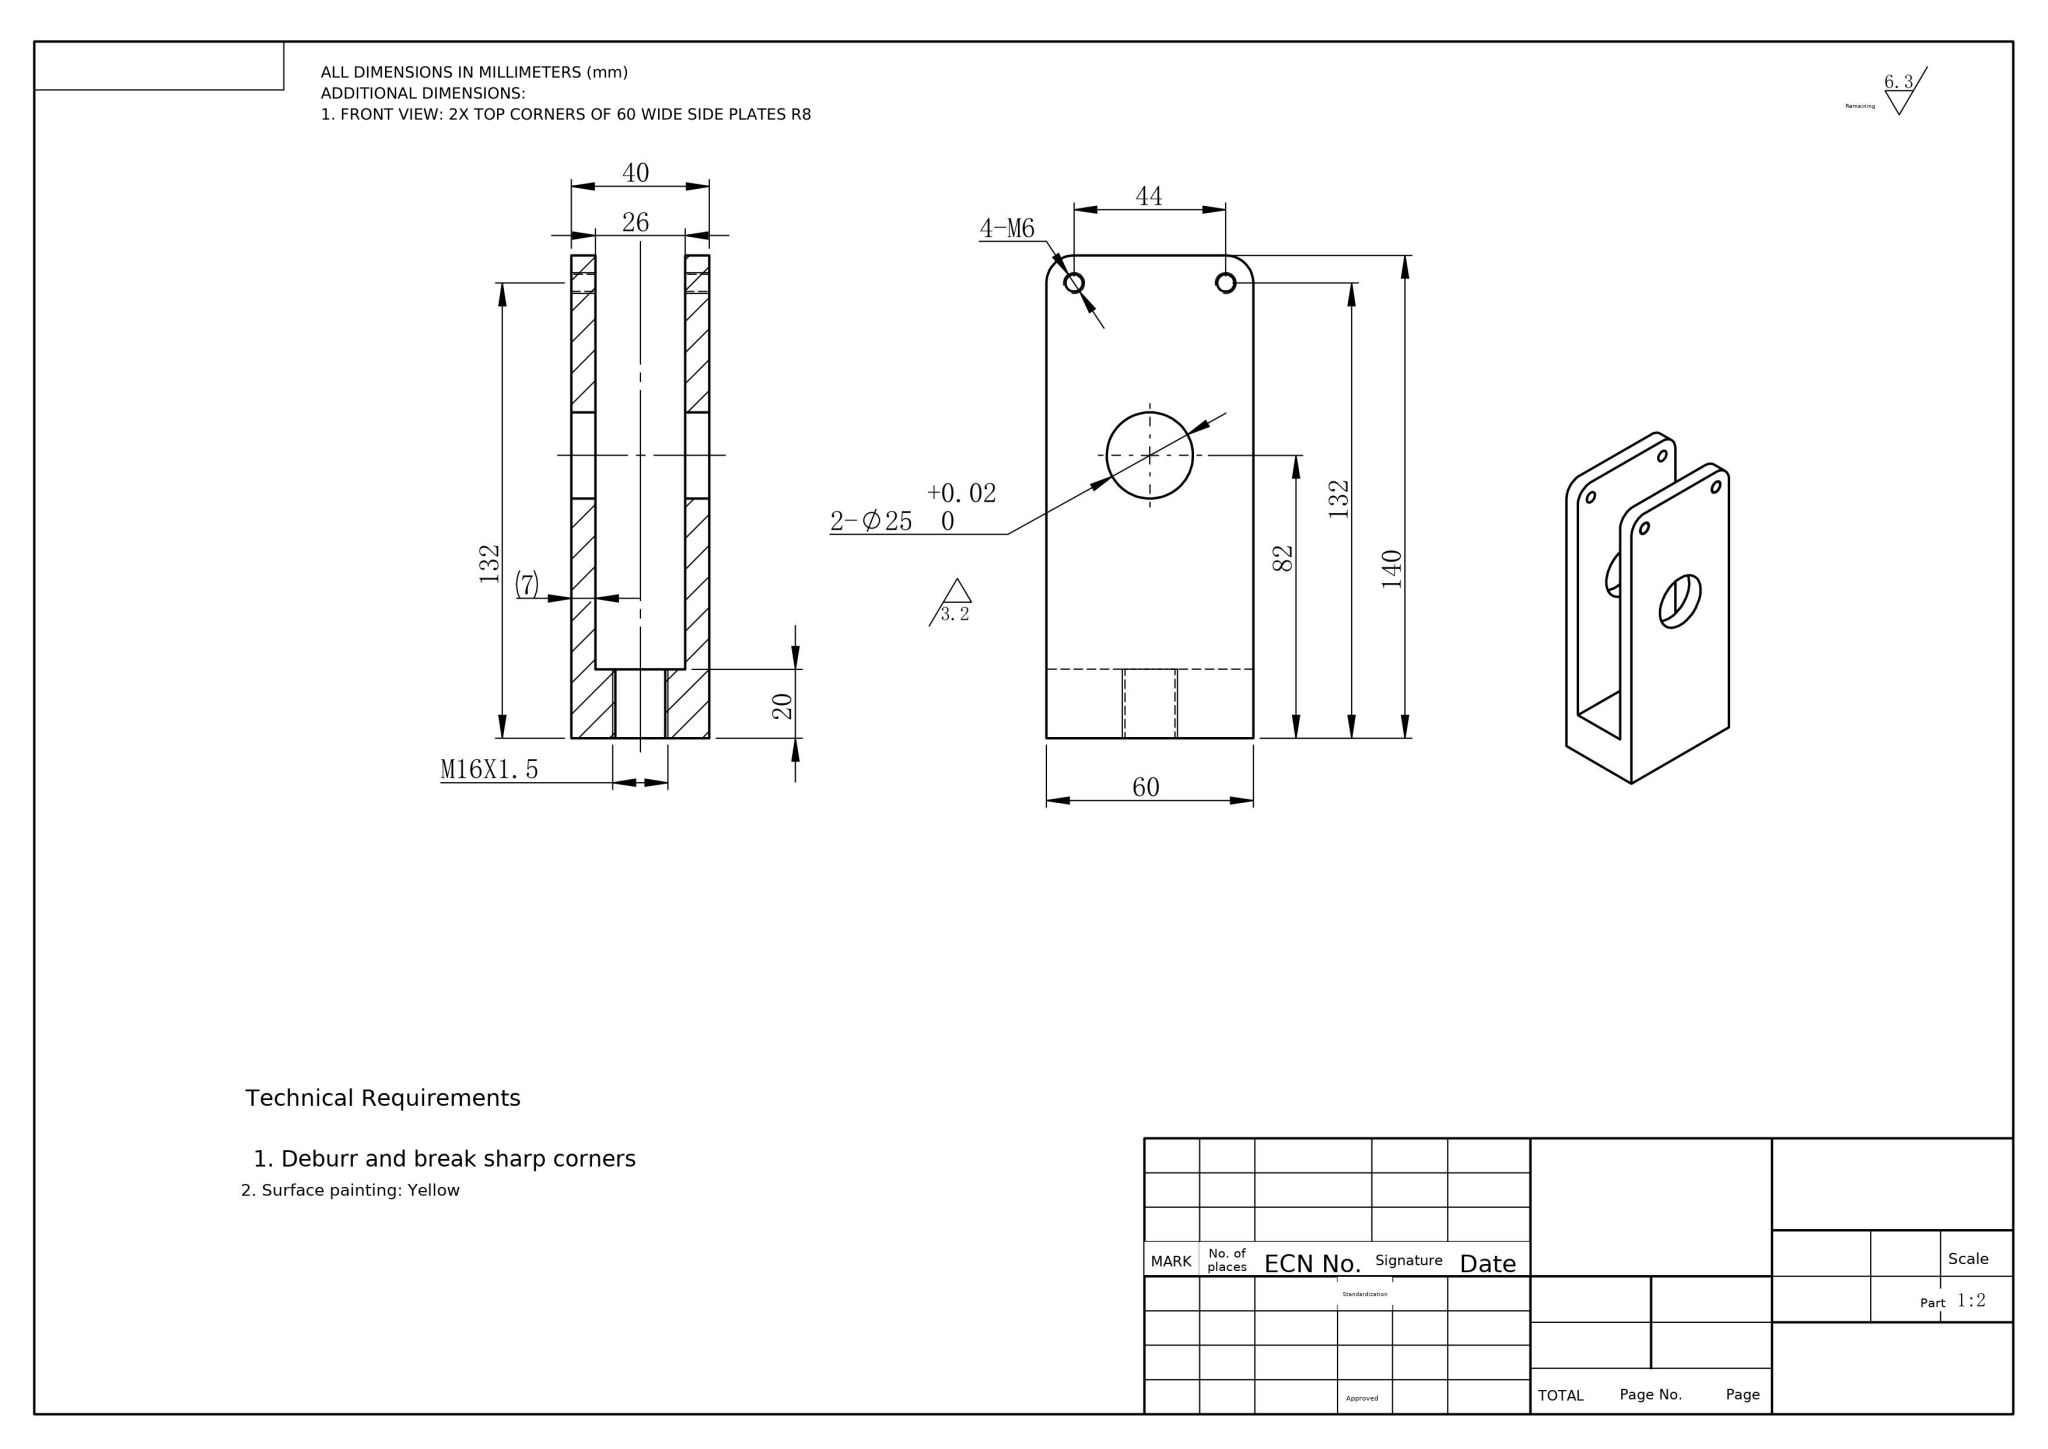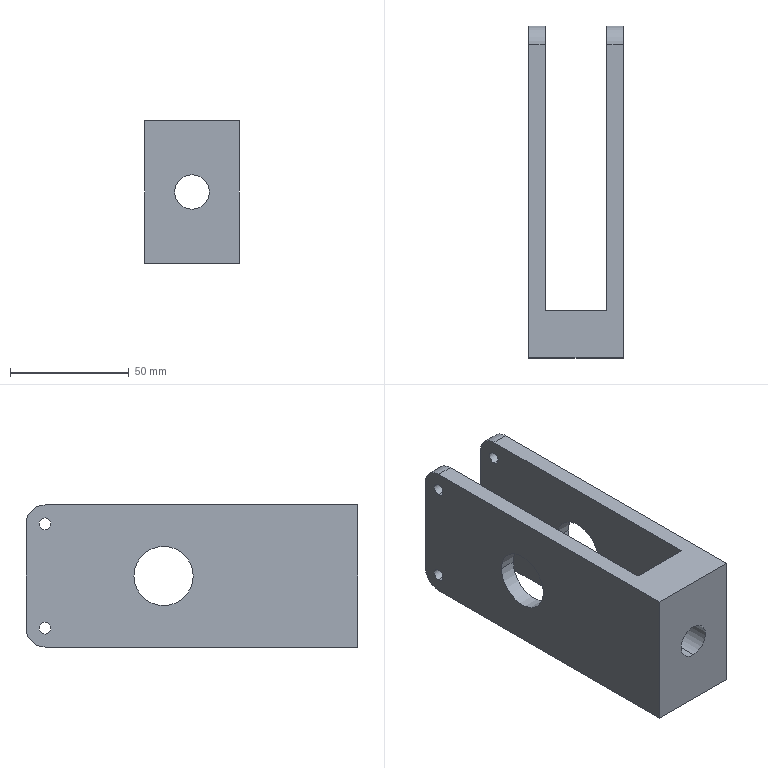Part | NX | mm | 1 solid | 28 faces | box 40 x 140 x 60 mm | volume 137691 mm3 | cylinder 18 | plane 10 | commonest cylinder face diameters 5 x8 25 x4 16 x4 14.5 x2